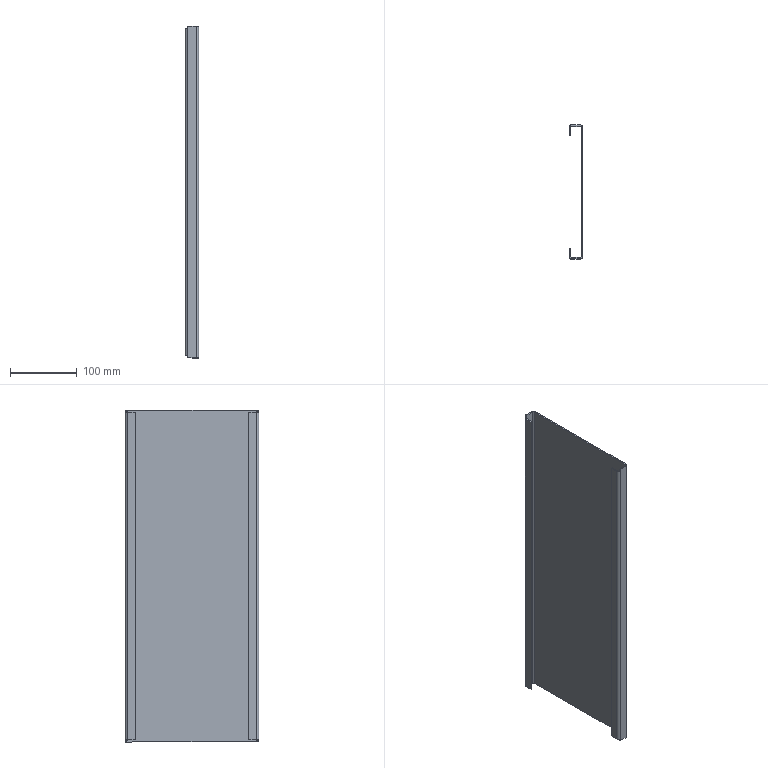Component | SolidWorks | BoxWelding-1_AuxiliaryPanel1-1 | 1 solid | 44 faces | volume 254298 mm3 | plane 34 | cylinder 10 | commonest cylinder face diameters 8 x6 4 x4